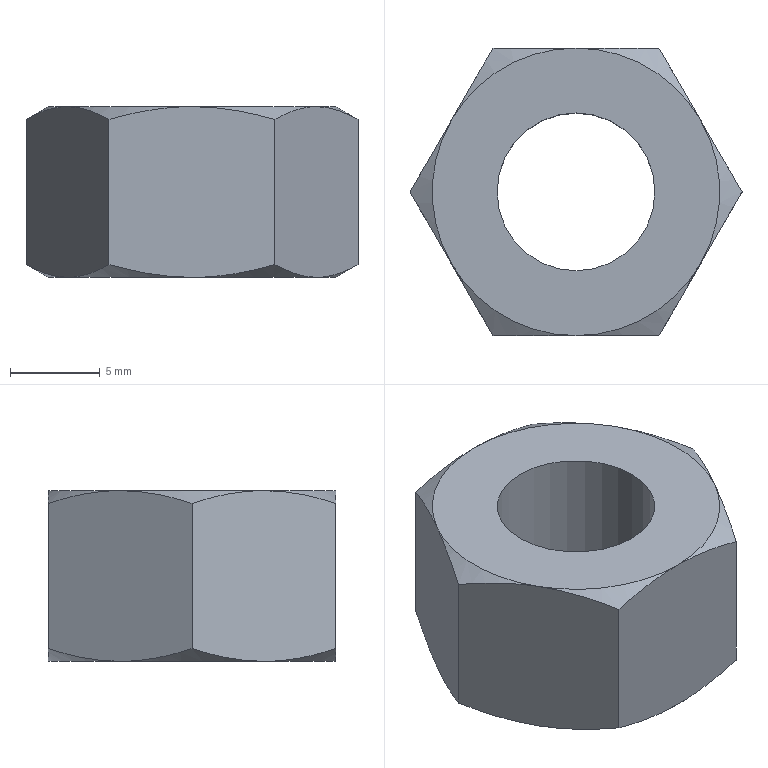Component | NX | GB-T41-2000_M10X1_5 | 1 solid | 21 faces | volume 1522 mm3 | cone 12 | plane 8 | cylinder 1 | commonest cylinder face diameters 8.782 x1